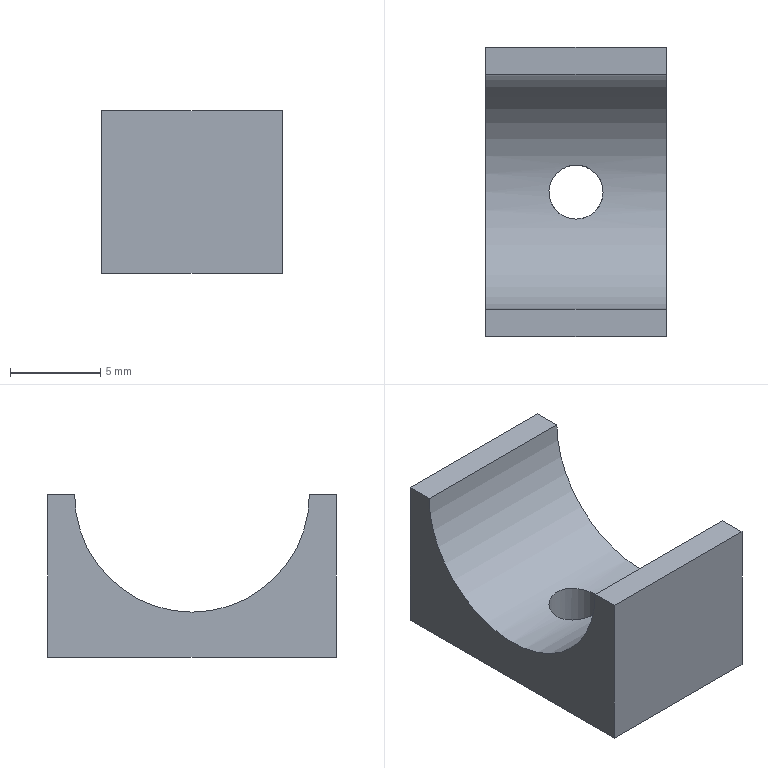Component | NX | 12A__27 | 1 solid | 9 faces | box 10 x 16 x 9 mm | volume 758 mm3 | plane 7 | cylinder 2 | commonest cylinder face diameters 13 x1 3 x1
STEP:
#1=CARTESIAN_POINT('',(0.,0.,0.));
#2=DIRECTION('',(0.,0.,1.));
#3=DIRECTION('',(1.,0.,0.));
#4=AXIS2_PLACEMENT_3D('',#1,#2,#3);
#5=CARTESIAN_POINT('',(34.022,103.108,73.432));
#6=VERTEX_POINT('',#5);
#7=CARTESIAN_POINT('',(44.022,103.108,73.432));
#8=VERTEX_POINT('',#7);
#9=CARTESIAN_POINT('',(34.022,103.108,73.432));
#10=DIRECTION('',(1.,0.,0.));
#11=VECTOR('',#10,1.);
#12=LINE('',#9,#11);
#13=CARTESIAN_POINT('',(34.022,109.608,73.432));
#14=DIRECTION('',(1.,0.,0.));
#15=DIRECTION('',(0.,0.,1.));
#16=AXIS2_PLACEMENT_3D('',#13,#14,#15);
#17=CYLINDRICAL_SURFACE('',#16,6.5);
#18=CARTESIAN_POINT('',(1.571,0.));
#19=DIRECTION('',(0.,1.));
#20=VECTOR('',#19,1.);
#21=LINE('',#18,#20);
#22=(GEOMETRIC_REPRESENTATION_CONTEXT(2)PARAMETRIC_REPRESENTATION_CONTEXT()REPRESENTATION_CONTEXT('',''));
#23=DEFINITIONAL_REPRESENTATION('',(#21),#22);
#24=PCURVE('',#17,#23);
#25=CARTESIAN_POINT('',(34.022,101.608,73.432));
#26=DIRECTION('',(0.,0.,-1.));
#27=DIRECTION('',(1.,0.,0.));
#28=AXIS2_PLACEMENT_3D('',#25,#26,#27);
#29=PLANE('',#28);
#30=CARTESIAN_POINT('',(0.,-1.5));
#31=DIRECTION('',(1.,0.));
#32=VECTOR('',#31,1.);
#33=LINE('',#30,#32);
#34=(GEOMETRIC_REPRESENTATION_CONTEXT(2)PARAMETRIC_REPRESENTATION_CONTEXT()REPRESENTATION_CONTEXT('',''));
#35=DEFINITIONAL_REPRESENTATION('',(#33),#34);
#36=PCURVE('',#29,#35);
#37=SURFACE_CURVE('',#12,(#24,#36),.PCURVE_S1.);
#38=EDGE_CURVE('',#6,#8,#37,.T.);
#39=ORIENTED_EDGE('',*,*,#38,.F.);
#40=CARTESIAN_POINT('',(34.022,116.108,73.432));
#41=VERTEX_POINT('',#40);
#42=CARTESIAN_POINT('',(34.022,109.608,73.432));
#43=DIRECTION('',(1.,0.,0.));
#44=DIRECTION('',(0.,-1.,0.));
#45=AXIS2_PLACEMENT_3D('',#42,#43,#44);
#46=CIRCLE('',#45,6.5);
#47=CARTESIAN_POINT('',(1.571,0.));
#48=DIRECTION('',(1.,0.));
#49=VECTOR('',#48,1.);
#50=LINE('',#47,#49);
#51=(GEOMETRIC_REPRESENTATION_CONTEXT(2)PARAMETRIC_REPRESENTATION_CONTEXT()REPRESENTATION_CONTEXT('',''));
#52=DEFINITIONAL_REPRESENTATION('',(#50),#51);
#53=PCURVE('',#17,#52);
#54=CARTESIAN_POINT('',(34.022,109.608,73.432));
#55=DIRECTION('',(1.,0.,0.));
#56=DIRECTION('',(0.,0.,1.));
#57=AXIS2_PLACEMENT_3D('',#54,#55,#56);
#58=PLANE('',#57);
#59=CARTESIAN_POINT('',(0.,0.));
#60=DIRECTION('',(0.,1.));
#61=AXIS2_PLACEMENT_2D('',#59,#60);
#62=CIRCLE('',#61,6.5);
#63=(GEOMETRIC_REPRESENTATION_CONTEXT(2)PARAMETRIC_REPRESENTATION_CONTEXT()REPRESENTATION_CONTEXT('',''));
#64=DEFINITIONAL_REPRESENTATION('',(#62),#63);
#65=PCURVE('',#58,#64);
#66=SURFACE_CURVE('',#46,(#53,#65),.PCURVE_S1.);
#67=EDGE_CURVE('',#6,#41,#66,.T.);
#68=ORIENTED_EDGE('',*,*,#67,.T.);
#69=CARTESIAN_POINT('',(44.022,116.108,73.432));
#70=VERTEX_POINT('',#69);
#71=CARTESIAN_POINT('',(34.022,116.108,73.432));
#72=DIRECTION('',(1.,0.,0.));
#73=VECTOR('',#72,1.);
#74=LINE('',#71,#73);
#75=CARTESIAN_POINT('',(4.712,0.));
#76=DIRECTION('',(0.,1.));
#77=VECTOR('',#76,1.);
#78=LINE('',#75,#77);
#79=(GEOMETRIC_REPRESENTATION_CONTEXT(2)PARAMETRIC_REPRESENTATION_CONTEXT()REPRESENTATION_CONTEXT('',''));
#80=DEFINITIONAL_REPRESENTATION('',(#78),#79);
#81=PCURVE('',#17,#80);
#82=CARTESIAN_POINT('',(34.022,116.108,73.432));
#83=DIRECTION('',(0.,0.,-1.));
#84=DIRECTION('',(1.,0.,0.));
#85=AXIS2_PLACEMENT_3D('',#82,#83,#84);
#86=PLANE('',#85);
#87=CARTESIAN_POINT('',(0.,0.));
#88=DIRECTION('',(1.,0.));
#89=VECTOR('',#88,1.);
#90=LINE('',#87,#89);
#91=(GEOMETRIC_REPRESENTATION_CONTEXT(2)PARAMETRIC_REPRESENTATION_CONTEXT()REPRESENTATION_CONTEXT('',''));
#92=DEFINITIONAL_REPRESENTATION('',(#90),#91);
#93=PCURVE('',#86,#92);
#94=SURFACE_CURVE('',#74,(#81,#93),.PCURVE_S1.);
#95=EDGE_CURVE('',#41,#70,#94,.T.);
#96=ORIENTED_EDGE('',*,*,#95,.T.);
#97=CARTESIAN_POINT('',(44.022,109.608,73.432));
#98=DIRECTION('',(1.,0.,0.));
#99=DIRECTION('',(0.,1.,0.));
#100=AXIS2_PLACEMENT_3D('',#97,#98,#99);
#101=CIRCLE('',#100,6.5);
#102=CARTESIAN_POINT('',(-1.571,10.));
#103=DIRECTION('',(1.,0.));
#104=VECTOR('',#103,1.);
#105=LINE('',#102,#104);
#106=(GEOMETRIC_REPRESENTATION_CONTEXT(2)PARAMETRIC_REPRESENTATION_CONTEXT()REPRESENTATION_CONTEXT('',''));
#107=DEFINITIONAL_REPRESENTATION('',(#105),#106);
#108=PCURVE('',#17,#107);
#109=CARTESIAN_POINT('',(44.022,109.608,73.432));
#110=DIRECTION('',(1.,0.,0.));
#111=DIRECTION('',(0.,0.,1.));
#112=AXIS2_PLACEMENT_3D('',#109,#110,#111);
#113=PLANE('',#112);
#114=CARTESIAN_POINT('',(0.,0.));
#115=DIRECTION('',(0.,-1.));
#116=AXIS2_PLACEMENT_2D('',#114,#115);
#117=CIRCLE('',#116,6.5);
#118=(GEOMETRIC_REPRESENTATION_CONTEXT(2)PARAMETRIC_REPRESENTATION_CONTEXT()REPRESENTATION_CONTEXT('',''));
#119=DEFINITIONAL_REPRESENTATION('',(#117),#118);
#120=PCURVE('',#113,#119);
#121=SURFACE_CURVE('',#101,(#108,#120),.PCURVE_S1.);
#122=EDGE_CURVE('',#8,#70,#121,.T.);
#123=ORIENTED_EDGE('',*,*,#122,.F.);
#124=EDGE_LOOP('',(#39,#68,#96,#123));
#125=FACE_BOUND('',#124,.F.);
#126=CARTESIAN_POINT('',(40.522,109.608,66.932));
#127=VERTEX_POINT('',#126);
#128=CARTESIAN_POINT('',(40.522,109.608,66.932));
#129=CARTESIAN_POINT('',(40.522,109.774,66.932));
#130=CARTESIAN_POINT('',(40.494,109.941,66.938));
#131=CARTESIAN_POINT('',(40.44,110.097,66.95));
#132=CARTESIAN_POINT('',(40.386,110.253,66.962));
#133=CARTESIAN_POINT('',(40.306,110.402,66.979));
#134=CARTESIAN_POINT('',(40.204,110.531,66.998));
#135=CARTESIAN_POINT('',(40.102,110.663,67.016));
#136=CARTESIAN_POINT('',(39.975,110.778,67.037));
#137=CARTESIAN_POINT('',(39.835,110.869,67.055));
#138=CARTESIAN_POINT('',(39.693,110.96,67.073));
#139=CARTESIAN_POINT('',(39.532,111.029,67.089));
#140=CARTESIAN_POINT('',(39.367,111.068,67.098));
#141=CARTESIAN_POINT('',(39.205,111.106,67.107));
#142=CARTESIAN_POINT('',(39.033,111.117,67.109));
#143=CARTESIAN_POINT('',(38.867,111.1,67.105));
#144=CARTESIAN_POINT('',(38.704,111.083,67.101));
#145=CARTESIAN_POINT('',(38.542,111.039,67.091));
#146=CARTESIAN_POINT('',(38.394,110.97,67.076));
#147=CARTESIAN_POINT('',(38.245,110.902,67.061));
#148=CARTESIAN_POINT('',(38.106,110.807,67.042));
#149=CARTESIAN_POINT('',(37.987,110.694,67.023));
#150=CARTESIAN_POINT('',(37.865,110.578,67.003));
#151=CARTESIAN_POINT('',(37.762,110.439,66.983));
#152=CARTESIAN_POINT('',(37.686,110.289,66.967));
#153=CARTESIAN_POINT('',(37.609,110.139,66.952));
#154=CARTESIAN_POINT('',(37.557,109.972,66.94));
#155=CARTESIAN_POINT('',(37.535,109.804,66.935));
#156=CARTESIAN_POINT('',(37.513,109.64,66.93));
#157=CARTESIAN_POINT('',(37.519,109.47,66.931));
#158=CARTESIAN_POINT('',(37.553,109.307,66.939));
#159=CARTESIAN_POINT('',(37.585,109.147,66.946));
#160=CARTESIAN_POINT('',(37.646,108.99,66.96));
#161=CARTESIAN_POINT('',(37.728,108.85,66.976));
#162=CARTESIAN_POINT('',(37.812,108.707,66.993));
#163=CARTESIAN_POINT('',(37.92,108.577,67.013));
#164=CARTESIAN_POINT('',(38.046,108.469,67.032));
#165=CARTESIAN_POINT('',(38.174,108.359,67.052));
#166=CARTESIAN_POINT('',(38.323,108.27,67.071));
#167=CARTESIAN_POINT('',(38.481,108.209,67.084));
#168=CARTESIAN_POINT('',(38.638,108.148,67.097));
#169=CARTESIAN_POINT('',(38.808,108.114,67.106));
#170=CARTESIAN_POINT('',(38.976,108.109,67.107));
#171=CARTESIAN_POINT('',(39.141,108.104,67.108));
#172=CARTESIAN_POINT('',(39.309,108.127,67.103));
#173=CARTESIAN_POINT('',(39.466,108.175,67.092));
#174=CARTESIAN_POINT('',(39.622,108.223,67.081));
#175=CARTESIAN_POINT('',(39.772,108.299,67.064));
#176=CARTESIAN_POINT('',(39.904,108.394,67.046));
#177=CARTESIAN_POINT('',(40.038,108.492,67.027));
#178=CARTESIAN_POINT('',(40.158,108.614,67.007));
#179=CARTESIAN_POINT('',(40.253,108.751,66.988));
#180=CARTESIAN_POINT('',(40.35,108.89,66.97));
#181=CARTESIAN_POINT('',(40.424,109.048,66.954));
#182=CARTESIAN_POINT('',(40.469,109.211,66.944));
#183=CARTESIAN_POINT('',(40.504,109.34,66.936));
#184=CARTESIAN_POINT('',(40.522,109.475,66.932));
#185=CARTESIAN_POINT('',(40.522,109.608,66.932));
#186=B_SPLINE_CURVE_WITH_KNOTS('',3,(#128,#129,#130,#131,#132,#133,#134,#135,#136,#137,#138,#139,#140,#141,#142,#143,#144,#145,#146,#147,#148,#149,#150,#151,#152,#153,#154,#155,#156,#157,#158,#159,#160,#161,#162,#163,#164,#165,#166,#167,#168,#169,#170,#171,#172,#173,#174,#175,#176,#177,#178,#179,#180,#181,#182,#183,#184,#185),.UNSPECIFIED.,.T.,.F.,(1,3,3,3,3,3,3,3,3,3,3,3,3,3,3,3,3,3,3,3,3,1),(-0.04234,0.,0.05275,0.1054,0.159,0.2132,0.2665,0.3187,0.3713,0.4252,0.4793,0.5321,0.5843,0.6373,0.6915,0.7453,0.7978,0.85,0.9034,0.9577,1.,1.053),.UNSPECIFIED.);
#187=CARTESIAN_POINT('',(3.142,6.5));
#188=CARTESIAN_POINT('',(3.147,6.5));
#189=CARTESIAN_POINT('',(3.158,6.497));
#190=CARTESIAN_POINT('',(3.175,6.486));
#191=CARTESIAN_POINT('',(3.191,6.467));
#192=CARTESIAN_POINT('',(3.207,6.44));
#193=CARTESIAN_POINT('',(3.223,6.406));
#194=CARTESIAN_POINT('',(3.238,6.365));
#195=CARTESIAN_POINT('',(3.253,6.317));
#196=CARTESIAN_POINT('',(3.267,6.262));
#197=CARTESIAN_POINT('',(3.281,6.201));
#198=CARTESIAN_POINT('',(3.293,6.135));
#199=CARTESIAN_POINT('',(3.306,6.062));
#200=CARTESIAN_POINT('',(3.317,5.983));
#201=CARTESIAN_POINT('',(3.328,5.9));
#202=CARTESIAN_POINT('',(3.337,5.813));
#203=CARTESIAN_POINT('',(3.346,5.721));
#204=CARTESIAN_POINT('',(3.353,5.625));
#205=CARTESIAN_POINT('',(3.36,5.526));
#206=CARTESIAN_POINT('',(3.365,5.424));
#207=CARTESIAN_POINT('',(3.369,5.321));
#208=CARTESIAN_POINT('',(3.372,5.215));
#209=CARTESIAN_POINT('',(3.374,5.108));
#210=CARTESIAN_POINT('',(3.375,5.));
#211=CARTESIAN_POINT('',(3.374,4.893));
#212=CARTESIAN_POINT('',(3.372,4.787));
#213=CARTESIAN_POINT('',(3.369,4.681));
#214=CARTESIAN_POINT('',(3.365,4.576));
#215=CARTESIAN_POINT('',(3.36,4.474));
#216=CARTESIAN_POINT('',(3.353,4.376));
#217=CARTESIAN_POINT('',(3.346,4.28));
#218=CARTESIAN_POINT('',(3.337,4.188));
#219=CARTESIAN_POINT('',(3.328,4.1));
#220=CARTESIAN_POINT('',(3.317,4.017));
#221=CARTESIAN_POINT('',(3.306,3.939));
#222=CARTESIAN_POINT('',(3.294,3.866));
#223=CARTESIAN_POINT('',(3.281,3.799));
#224=CARTESIAN_POINT('',(3.267,3.738));
#225=CARTESIAN_POINT('',(3.253,3.683));
#226=CARTESIAN_POINT('',(3.238,3.635));
#227=CARTESIAN_POINT('',(3.223,3.594));
#228=CARTESIAN_POINT('',(3.207,3.56));
#229=CARTESIAN_POINT('',(3.191,3.533));
#230=CARTESIAN_POINT('',(3.175,3.514));
#231=CARTESIAN_POINT('',(3.158,3.503));
#232=CARTESIAN_POINT('',(3.142,3.499));
#233=CARTESIAN_POINT('',(3.125,3.503));
#234=CARTESIAN_POINT('',(3.109,3.514));
#235=CARTESIAN_POINT('',(3.092,3.533));
#236=CARTESIAN_POINT('',(3.076,3.56));
#237=CARTESIAN_POINT('',(3.061,3.594));
#238=CARTESIAN_POINT('',(3.045,3.635));
#239=CARTESIAN_POINT('',(3.031,3.683));
#240=CARTESIAN_POINT('',(3.016,3.737));
#241=CARTESIAN_POINT('',(3.003,3.798));
#242=CARTESIAN_POINT('',(2.99,3.865));
#243=CARTESIAN_POINT('',(2.978,3.938));
#244=CARTESIAN_POINT('',(2.966,4.016));
#245=CARTESIAN_POINT('',(2.956,4.099));
#246=CARTESIAN_POINT('',(2.946,4.187));
#247=CARTESIAN_POINT('',(2.938,4.279));
#248=CARTESIAN_POINT('',(2.93,4.375));
#249=CARTESIAN_POINT('',(2.924,4.473));
#250=CARTESIAN_POINT('',(2.918,4.575));
#251=CARTESIAN_POINT('',(2.914,4.679));
#252=CARTESIAN_POINT('',(2.911,4.785));
#253=CARTESIAN_POINT('',(2.909,4.892));
#254=CARTESIAN_POINT('',(2.909,4.999));
#255=CARTESIAN_POINT('',(2.909,5.106));
#256=CARTESIAN_POINT('',(2.911,5.213));
#257=CARTESIAN_POINT('',(2.914,5.319));
#258=CARTESIAN_POINT('',(2.918,5.423));
#259=CARTESIAN_POINT('',(2.923,5.524));
#260=CARTESIAN_POINT('',(2.93,5.624));
#261=CARTESIAN_POINT('',(2.937,5.72));
#262=CARTESIAN_POINT('',(2.946,5.812));
#263=CARTESIAN_POINT('',(2.956,5.899));
#264=CARTESIAN_POINT('',(2.966,5.982));
#265=CARTESIAN_POINT('',(2.977,6.061));
#266=CARTESIAN_POINT('',(2.99,6.134));
#267=CARTESIAN_POINT('',(3.003,6.201));
#268=CARTESIAN_POINT('',(3.016,6.262));
#269=CARTESIAN_POINT('',(3.03,6.316));
#270=CARTESIAN_POINT('',(3.045,6.364));
#271=CARTESIAN_POINT('',(3.06,6.406));
#272=CARTESIAN_POINT('',(3.076,6.44));
#273=CARTESIAN_POINT('',(3.092,6.466));
#274=CARTESIAN_POINT('',(3.109,6.486));
#275=CARTESIAN_POINT('',(3.125,6.497));
#276=CARTESIAN_POINT('',(3.136,6.5));
#277=CARTESIAN_POINT('',(3.142,6.5));
#278=B_SPLINE_CURVE_WITH_KNOTS('',3,(#187,#188,#189,#190,#191,#192,#193,#194,#195,#196,#197,#198,#199,#200,#201,#202,#203,#204,#205,#206,#207,#208,#209,#210,#211,#212,#213,#214,#215,#216,#217,#218,#219,#220,#221,#222,#223,#224,#225,#226,#227,#228,#229,#230,#231,#232,#233,#234,#235,#236,#237,#238,#239,#240,#241,#242,#243,#244,#245,#246,#247,#248,#249,#250,#251,#252,#253,#254,#255,#256,#257,#258,#259,#260,#261,#262,#263,#264,#265,#266,#267,#268,#269,#270,#271,#272,#273,#274,#275,#276,#277),.UNSPECIFIED.,.T.,.F.,(4,1,1,1,1,1,1,1,1,1,1,1,1,1,1,1,1,1,1,1,1,1,1,1,1,1,1,1,1,1,1,1,1,1,1,1,1,1,1,1,1,1,1,1,1,1,1,1,1,1,1,1,1,1,1,1,1,1,1,1,1,1,1,1,1,1,1,1,1,1,1,1,1,1,1,1,1,1,1,1,1,1,1,1,1,1,1,1,4),(0.,0.01136,0.02273,0.03409,0.04545,0.05682,0.06818,0.07955,0.09091,0.1023,0.1136,0.125,0.1364,0.1477,0.1591,0.1705,0.1818,0.1932,0.2045,0.2159,0.2273,0.2386,0.25,0.2614,0.2727,0.2841,0.2955,0.3068,0.3182,0.3295,0.3409,0.3523,0.3636,0.375,0.3864,0.3977,0.4091,0.4205,0.4318,0.4432,0.4545,0.4659,0.4773,0.4886,0.5,0.5114,0.5227,0.5341,0.5455,0.5568,0.5682,0.5795,0.5909,0.6023,0.6136,0.625,0.6364,0.6477,0.6591,0.6705,0.6818,0.6932,0.7045,0.7159,0.7273,0.7386,0.75,0.7614,0.7727,0.7841,0.7955,0.8068,0.8182,0.8295,0.8409,0.8523,0.8636,0.875,0.8864,0.8977,0.9091,0.9205,0.9318,0.9432,0.9545,0.9659,0.9773,0.9886,1.),.QUASI_UNIFORM_KNOTS.);
#279=(GEOMETRIC_REPRESENTATION_CONTEXT(2)PARAMETRIC_REPRESENTATION_CONTEXT()REPRESENTATION_CONTEXT('',''));
#280=DEFINITIONAL_REPRESENTATION('',(#278),#279);
#281=PCURVE('',#17,#280);
#282=CARTESIAN_POINT('',(39.022,109.608,74.432));
#283=DIRECTION('',(0.,0.,-1.));
#284=DIRECTION('',(1.,0.,0.));
#285=AXIS2_PLACEMENT_3D('',#282,#283,#284);
#286=CYLINDRICAL_SURFACE('',#285,1.5);
#287=CARTESIAN_POINT('',(6.283,7.5));
#288=CARTESIAN_POINT('',(6.259,7.5));
#289=CARTESIAN_POINT('',(6.212,7.499));
#290=CARTESIAN_POINT('',(6.14,7.497));
#291=CARTESIAN_POINT('',(6.068,7.492));
#292=CARTESIAN_POINT('',(5.997,7.486));
#293=CARTESIAN_POINT('',(5.926,7.479));
#294=CARTESIAN_POINT('',(5.854,7.47));
#295=CARTESIAN_POINT('',(5.783,7.46));
#296=CARTESIAN_POINT('',(5.711,7.449));
#297=CARTESIAN_POINT('',(5.64,7.438));
#298=CARTESIAN_POINT('',(5.569,7.425));
#299=CARTESIAN_POINT('',(5.498,7.413));
#300=CARTESIAN_POINT('',(5.427,7.4));
#301=CARTESIAN_POINT('',(5.355,7.388));
#302=CARTESIAN_POINT('',(5.284,7.376));
#303=CARTESIAN_POINT('',(5.213,7.365));
#304=CARTESIAN_POINT('',(5.142,7.355));
#305=CARTESIAN_POINT('',(5.07,7.346));
#306=CARTESIAN_POINT('',(4.999,7.338));
#307=CARTESIAN_POINT('',(4.928,7.332));
#308=CARTESIAN_POINT('',(4.856,7.328));
#309=CARTESIAN_POINT('',(4.784,7.325));
#310=CARTESIAN_POINT('',(4.713,7.324));
#311=CARTESIAN_POINT('',(4.641,7.325));
#312=CARTESIAN_POINT('',(4.57,7.328));
#313=CARTESIAN_POINT('',(4.498,7.332));
#314=CARTESIAN_POINT('',(4.426,7.339));
#315=CARTESIAN_POINT('',(4.355,7.346));
#316=CARTESIAN_POINT('',(4.283,7.355));
#317=CARTESIAN_POINT('',(4.212,7.365));
#318=CARTESIAN_POINT('',(4.141,7.376));
#319=CARTESIAN_POINT('',(4.07,7.388));
#320=CARTESIAN_POINT('',(3.998,7.4));
#321=CARTESIAN_POINT('',(3.927,7.413));
#322=CARTESIAN_POINT('',(3.856,7.425));
#323=CARTESIAN_POINT('',(3.785,7.437));
#324=CARTESIAN_POINT('',(3.714,7.449));
#325=CARTESIAN_POINT('',(3.642,7.46));
#326=CARTESIAN_POINT('',(3.571,7.47));
#327=CARTESIAN_POINT('',(3.5,7.479));
#328=CARTESIAN_POINT('',(3.428,7.486));
#329=CARTESIAN_POINT('',(3.357,7.492));
#330=CARTESIAN_POINT('',(3.285,7.497));
#331=CARTESIAN_POINT('',(3.214,7.499));
#332=CARTESIAN_POINT('',(3.142,7.5));
#333=CARTESIAN_POINT('',(3.07,7.499));
#334=CARTESIAN_POINT('',(2.999,7.497));
#335=CARTESIAN_POINT('',(2.927,7.492));
#336=CARTESIAN_POINT('',(2.856,7.486));
#337=CARTESIAN_POINT('',(2.784,7.479));
#338=CARTESIAN_POINT('',(2.713,7.47));
#339=CARTESIAN_POINT('',(2.641,7.46));
#340=CARTESIAN_POINT('',(2.57,7.449));
#341=CARTESIAN_POINT('',(2.499,7.438));
#342=CARTESIAN_POINT('',(2.428,7.425));
#343=CARTESIAN_POINT('',(2.357,7.413));
#344=CARTESIAN_POINT('',(2.285,7.4));
#345=CARTESIAN_POINT('',(2.215,7.388));
#346=CARTESIAN_POINT('',(2.143,7.376));
#347=CARTESIAN_POINT('',(2.072,7.365));
#348=CARTESIAN_POINT('',(2.,7.355));
#349=CARTESIAN_POINT('',(1.929,7.346));
#350=CARTESIAN_POINT('',(1.858,7.339));
#351=CARTESIAN_POINT('',(1.786,7.332));
#352=CARTESIAN_POINT('',(1.715,7.328));
#353=CARTESIAN_POINT('',(1.643,7.325));
#354=CARTESIAN_POINT('',(1.572,7.324));
#355=CARTESIAN_POINT('',(1.5,7.325));
#356=CARTESIAN_POINT('',(1.428,7.328));
#357=CARTESIAN_POINT('',(1.357,7.332));
#358=CARTESIAN_POINT('',(1.285,7.338));
#359=CARTESIAN_POINT('',(1.214,7.346));
#360=CARTESIAN_POINT('',(1.142,7.355));
#361=CARTESIAN_POINT('',(1.071,7.365));
#362=CARTESIAN_POINT('',(0.9995,7.376));
#363=CARTESIAN_POINT('',(0.9286,7.388));
#364=CARTESIAN_POINT('',(0.8575,7.4));
#365=CARTESIAN_POINT('',(0.7862,7.413));
#366=CARTESIAN_POINT('',(0.7149,7.425));
#367=CARTESIAN_POINT('',(0.6436,7.437));
#368=CARTESIAN_POINT('',(0.5728,7.449));
#369=CARTESIAN_POINT('',(0.5015,7.46));
#370=CARTESIAN_POINT('',(0.43,7.47));
#371=CARTESIAN_POINT('',(0.3585,7.479));
#372=CARTESIAN_POINT('',(0.2872,7.486));
#373=CARTESIAN_POINT('',(0.2157,7.492));
#374=CARTESIAN_POINT('',(0.1438,7.497));
#375=CARTESIAN_POINT('',(0.07178,7.499));
#376=CARTESIAN_POINT('',(0.02388,7.5));
#377=CARTESIAN_POINT('',(0.,7.5));
#378=B_SPLINE_CURVE_WITH_KNOTS('',3,(#287,#288,#289,#290,#291,#292,#293,#294,#295,#296,#297,#298,#299,#300,#301,#302,#303,#304,#305,#306,#307,#308,#309,#310,#311,#312,#313,#314,#315,#316,#317,#318,#319,#320,#321,#322,#323,#324,#325,#326,#327,#328,#329,#330,#331,#332,#333,#334,#335,#336,#337,#338,#339,#340,#341,#342,#343,#344,#345,#346,#347,#348,#349,#350,#351,#352,#353,#354,#355,#356,#357,#358,#359,#360,#361,#362,#363,#364,#365,#366,#367,#368,#369,#370,#371,#372,#373,#374,#375,#376,#377),.UNSPECIFIED.,.F.,.F.,(4,1,1,1,1,1,1,1,1,1,1,1,1,1,1,1,1,1,1,1,1,1,1,1,1,1,1,1,1,1,1,1,1,1,1,1,1,1,1,1,1,1,1,1,1,1,1,1,1,1,1,1,1,1,1,1,1,1,1,1,1,1,1,1,1,1,1,1,1,1,1,1,1,1,1,1,1,1,1,1,1,1,1,1,1,1,1,1,4),(0.,0.01136,0.02273,0.03409,0.04545,0.05682,0.06818,0.07955,0.09091,0.1023,0.1136,0.125,0.1364,0.1477,0.1591,0.1705,0.1818,0.1932,0.2045,0.2159,0.2273,0.2386,0.25,0.2614,0.2727,0.2841,0.2955,0.3068,0.3182,0.3295,0.3409,0.3523,0.3636,0.375,0.3864,0.3977,0.4091,0.4205,0.4318,0.4432,0.4545,0.4659,0.4773,0.4886,0.5,0.5114,0.5227,0.5341,0.5455,0.5568,0.5682,0.5795,0.5909,0.6023,0.6136,0.625,0.6364,0.6477,0.6591,0.6705,0.6818,0.6932,0.7045,0.7159,0.7273,0.7386,0.75,0.7614,0.7727,0.7841,0.7955,0.8068,0.8182,0.8295,0.8409,0.8523,0.8636,0.875,0.8864,0.8977,0.9091,0.9205,0.9318,0.9432,0.9545,0.9659,0.9773,0.9886,1.),.QUASI_UNIFORM_KNOTS.);
#379=(GEOMETRIC_REPRESENTATION_CONTEXT(2)PARAMETRIC_REPRESENTATION_CONTEXT()REPRESENTATION_CONTEXT('',''));
#380=DEFINITIONAL_REPRESENTATION('',(#378),#379);
#381=PCURVE('',#286,#380);
#382=SURFACE_CURVE('',#186,(#281,#381),.PCURVE_S1.);
#383=EDGE_CURVE('',#127,#127,#382,.T.);
#384=ORIENTED_EDGE('',*,*,#383,.T.);
#385=EDGE_LOOP('',(#384));
#386=FACE_BOUND('',#385,.F.);
#387=ADVANCED_FACE('',(#125,#386),#17,.F.);
#388=CARTESIAN_POINT('',(44.022,101.608,64.432));
#389=VERTEX_POINT('',#388);
#390=CARTESIAN_POINT('',(44.022,101.608,73.432));
#391=VERTEX_POINT('',#390);
#392=CARTESIAN_POINT('',(44.022,101.608,64.432));
#393=DIRECTION('',(0.,0.,1.));
#394=VECTOR('',#393,1.);
#395=LINE('',#392,#394);
#396=CARTESIAN_POINT('',(34.022,101.608,64.432));
#397=DIRECTION('',(0.,1.,0.));
#398=DIRECTION('',(0.,0.,-1.));
#399=AXIS2_PLACEMENT_3D('',#396,#397,#398);
#400=PLANE('',#399);
#401=CARTESIAN_POINT('',(0.,-10.));
#402=DIRECTION('',(-1.,0.));
#403=VECTOR('',#402,1.);
#404=LINE('',#401,#403);
#405=(GEOMETRIC_REPRESENTATION_CONTEXT(2)PARAMETRIC_REPRESENTATION_CONTEXT()REPRESENTATION_CONTEXT('',''));
#406=DEFINITIONAL_REPRESENTATION('',(#404),#405);
#407=PCURVE('',#400,#406);
#408=CARTESIAN_POINT('',(-9.,8.));
#409=DIRECTION('',(1.,0.));
#410=VECTOR('',#409,1.);
#411=LINE('',#408,#410);
#412=(GEOMETRIC_REPRESENTATION_CONTEXT(2)PARAMETRIC_REPRESENTATION_CONTEXT()REPRESENTATION_CONTEXT('',''));
#413=DEFINITIONAL_REPRESENTATION('',(#411),#412);
#414=PCURVE('',#113,#413);
#415=SURFACE_CURVE('',#395,(#407,#414),.PCURVE_S1.);
#416=EDGE_CURVE('',#389,#391,#415,.T.);
#417=ORIENTED_EDGE('',*,*,#416,.T.);
#418=CARTESIAN_POINT('',(34.022,101.608,73.432));
#419=VERTEX_POINT('',#418);
#420=CARTESIAN_POINT('',(34.022,101.608,73.432));
#421=DIRECTION('',(1.,0.,0.));
#422=VECTOR('',#421,1.);
#423=LINE('',#420,#422);
#424=CARTESIAN_POINT('',(-9.,0.));
#425=DIRECTION('',(0.,-1.));
#426=VECTOR('',#425,1.);
#427=LINE('',#424,#426);
#428=(GEOMETRIC_REPRESENTATION_CONTEXT(2)PARAMETRIC_REPRESENTATION_CONTEXT()REPRESENTATION_CONTEXT('',''));
#429=DEFINITIONAL_REPRESENTATION('',(#427),#428);
#430=PCURVE('',#400,#429);
#431=CARTESIAN_POINT('',(0.,0.));
#432=DIRECTION('',(1.,0.));
#433=VECTOR('',#432,1.);
#434=LINE('',#431,#433);
#435=(GEOMETRIC_REPRESENTATION_CONTEXT(2)PARAMETRIC_REPRESENTATION_CONTEXT()REPRESENTATION_CONTEXT('',''));
#436=DEFINITIONAL_REPRESENTATION('',(#434),#435);
#437=PCURVE('',#29,#436);
#438=SURFACE_CURVE('',#423,(#430,#437),.PCURVE_S1.);
#439=EDGE_CURVE('',#419,#391,#438,.T.);
#440=ORIENTED_EDGE('',*,*,#439,.F.);
#441=CARTESIAN_POINT('',(34.022,101.608,64.432));
#442=VERTEX_POINT('',#441);
#443=CARTESIAN_POINT('',(34.022,101.608,64.432));
#444=DIRECTION('',(0.,0.,1.));
#445=VECTOR('',#444,1.);
#446=LINE('',#443,#445);
#447=CARTESIAN_POINT('',(0.,0.));
#448=DIRECTION('',(-1.,0.));
#449=VECTOR('',#448,1.);
#450=LINE('',#447,#449);
#451=(GEOMETRIC_REPRESENTATION_CONTEXT(2)PARAMETRIC_REPRESENTATION_CONTEXT()REPRESENTATION_CONTEXT('',''));
#452=DEFINITIONAL_REPRESENTATION('',(#450),#451);
#453=PCURVE('',#400,#452);
#454=CARTESIAN_POINT('',(-9.,8.));
#455=DIRECTION('',(1.,0.));
#456=VECTOR('',#455,1.);
#457=LINE('',#454,#456);
#458=(GEOMETRIC_REPRESENTATION_CONTEXT(2)PARAMETRIC_REPRESENTATION_CONTEXT()REPRESENTATION_CONTEXT('',''));
#459=DEFINITIONAL_REPRESENTATION('',(#457),#458);
#460=PCURVE('',#58,#459);
#461=SURFACE_CURVE('',#446,(#453,#460),.PCURVE_S1.);
#462=EDGE_CURVE('',#442,#419,#461,.T.);
#463=ORIENTED_EDGE('',*,*,#462,.F.);
#464=CARTESIAN_POINT('',(34.022,101.608,64.432));
#465=DIRECTION('',(1.,0.,0.));
#466=VECTOR('',#465,1.);
#467=LINE('',#464,#466);
#468=CARTESIAN_POINT('',(0.,0.));
#469=DIRECTION('',(0.,-1.));
#470=VECTOR('',#469,1.);
#471=LINE('',#468,#470);
#472=(GEOMETRIC_REPRESENTATION_CONTEXT(2)PARAMETRIC_REPRESENTATION_CONTEXT()REPRESENTATION_CONTEXT('',''));
#473=DEFINITIONAL_REPRESENTATION('',(#471),#472);
#474=PCURVE('',#400,#473);
#475=CARTESIAN_POINT('',(34.022,117.608,64.432));
#476=DIRECTION('',(0.,0.,1.));
#477=DIRECTION('',(-1.,0.,0.));
#478=AXIS2_PLACEMENT_3D('',#475,#476,#477);
#479=PLANE('',#478);
#480=CARTESIAN_POINT('',(0.,16.));
#481=DIRECTION('',(-1.,0.));
#482=VECTOR('',#481,1.);
#483=LINE('',#480,#482);
#484=(GEOMETRIC_REPRESENTATION_CONTEXT(2)PARAMETRIC_REPRESENTATION_CONTEXT()REPRESENTATION_CONTEXT('',''));
#485=DEFINITIONAL_REPRESENTATION('',(#483),#484);
#486=PCURVE('',#479,#485);
#487=SURFACE_CURVE('',#467,(#474,#486),.PCURVE_S1.);
#488=EDGE_CURVE('',#442,#389,#487,.T.);
#489=ORIENTED_EDGE('',*,*,#488,.T.);
#490=EDGE_LOOP('',(#417,#440,#463,#489));
#491=FACE_BOUND('',#490,.T.);
#492=ADVANCED_FACE('',(#491),#400,.F.);
#493=CARTESIAN_POINT('',(44.022,101.608,73.432));
#494=DIRECTION('',(0.,1.,0.));
#495=VECTOR('',#494,1.);
#496=LINE('',#493,#495);
#497=CARTESIAN_POINT('',(10.,0.));
#498=DIRECTION('',(0.,-1.));
#499=VECTOR('',#498,1.);
#500=LINE('',#497,#499);
#501=(GEOMETRIC_REPRESENTATION_CONTEXT(2)PARAMETRIC_REPRESENTATION_CONTEXT()REPRESENTATION_CONTEXT('',''));
#502=DEFINITIONAL_REPRESENTATION('',(#500),#501);
#503=PCURVE('',#29,#502);
#504=CARTESIAN_POINT('',(0.,8.));
#505=DIRECTION('',(0.,-1.));
#506=VECTOR('',#505,1.);
#507=LINE('',#504,#506);
#508=(GEOMETRIC_REPRESENTATION_CONTEXT(2)PARAMETRIC_REPRESENTATION_CONTEXT()REPRESENTATION_CONTEXT('',''));
#509=DEFINITIONAL_REPRESENTATION('',(#507),#508);
#510=PCURVE('',#113,#509);
#511=SURFACE_CURVE('',#496,(#503,#510),.PCURVE_S1.);
#512=EDGE_CURVE('',#391,#8,#511,.T.);
#513=ORIENTED_EDGE('',*,*,#512,.T.);
#514=ORIENTED_EDGE('',*,*,#38,.F.);
#515=CARTESIAN_POINT('',(34.022,101.608,73.432));
#516=DIRECTION('',(0.,1.,0.));
#517=VECTOR('',#516,1.);
#518=LINE('',#515,#517);
#519=CARTESIAN_POINT('',(0.,0.));
#520=DIRECTION('',(0.,-1.));
#521=VECTOR('',#520,1.);
#522=LINE('',#519,#521);
#523=(GEOMETRIC_REPRESENTATION_CONTEXT(2)PARAMETRIC_REPRESENTATION_CONTEXT()REPRESENTATION_CONTEXT('',''));
#524=DEFINITIONAL_REPRESENTATION('',(#522),#523);
#525=PCURVE('',#29,#524);
#526=CARTESIAN_POINT('',(0.,8.));
#527=DIRECTION('',(0.,-1.));
#528=VECTOR('',#527,1.);
#529=LINE('',#526,#528);
#530=(GEOMETRIC_REPRESENTATION_CONTEXT(2)PARAMETRIC_REPRESENTATION_CONTEXT()REPRESENTATION_CONTEXT('',''));
#531=DEFINITIONAL_REPRESENTATION('',(#529),#530);
#532=PCURVE('',#58,#531);
#533=SURFACE_CURVE('',#518,(#525,#532),.PCURVE_S1.);
#534=EDGE_CURVE('',#419,#6,#533,.T.);
#535=ORIENTED_EDGE('',*,*,#534,.F.);
#536=ORIENTED_EDGE('',*,*,#439,.T.);
#537=EDGE_LOOP('',(#513,#514,#535,#536));
#538=FACE_BOUND('',#537,.T.);
#539=ADVANCED_FACE('',(#538),#29,.F.);
#540=CARTESIAN_POINT('',(44.022,117.608,73.432));
#541=VERTEX_POINT('',#540);
#542=CARTESIAN_POINT('',(44.022,116.108,73.432));
#543=DIRECTION('',(0.,1.,0.));
#544=VECTOR('',#543,1.);
#545=LINE('',#542,#544);
#546=CARTESIAN_POINT('',(10.,0.));
#547=DIRECTION('',(0.,-1.));
#548=VECTOR('',#547,1.);
#549=LINE('',#546,#548);
#550=(GEOMETRIC_REPRESENTATION_CONTEXT(2)PARAMETRIC_REPRESENTATION_CONTEXT()REPRESENTATION_CONTEXT('',''));
#551=DEFINITIONAL_REPRESENTATION('',(#549),#550);
#552=PCURVE('',#86,#551);
#553=CARTESIAN_POINT('',(0.,-6.5));
#554=DIRECTION('',(0.,-1.));
#555=VECTOR('',#554,1.);
#556=LINE('',#553,#555);
#557=(GEOMETRIC_REPRESENTATION_CONTEXT(2)PARAMETRIC_REPRESENTATION_CONTEXT()REPRESENTATION_CONTEXT('',''));
#558=DEFINITIONAL_REPRESENTATION('',(#556),#557);
#559=PCURVE('',#113,#558);
#560=SURFACE_CURVE('',#545,(#552,#559),.PCURVE_S1.);
#561=EDGE_CURVE('',#70,#541,#560,.T.);
#562=ORIENTED_EDGE('',*,*,#561,.T.);
#563=CARTESIAN_POINT('',(34.022,117.608,73.432));
#564=VERTEX_POINT('',#563);
#565=CARTESIAN_POINT('',(34.022,117.608,73.432));
#566=DIRECTION('',(1.,0.,0.));
#567=VECTOR('',#566,1.);
#568=LINE('',#565,#567);
#569=CARTESIAN_POINT('',(0.,-1.5));
#570=DIRECTION('',(1.,0.));
#571=VECTOR('',#570,1.);
#572=LINE('',#569,#571);
#573=(GEOMETRIC_REPRESENTATION_CONTEXT(2)PARAMETRIC_REPRESENTATION_CONTEXT()REPRESENTATION_CONTEXT('',''));
#574=DEFINITIONAL_REPRESENTATION('',(#572),#573);
#575=PCURVE('',#86,#574);
#576=CARTESIAN_POINT('',(34.022,117.608,73.432));
#577=DIRECTION('',(0.,-1.,0.));
#578=DIRECTION('',(0.,0.,1.));
#579=AXIS2_PLACEMENT_3D('',#576,#577,#578);
#580=PLANE('',#579);
#581=CARTESIAN_POINT('',(0.,0.));
#582=DIRECTION('',(0.,-1.));
#583=VECTOR('',#582,1.);
#584=LINE('',#581,#583);
#585=(GEOMETRIC_REPRESENTATION_CONTEXT(2)PARAMETRIC_REPRESENTATION_CONTEXT()REPRESENTATION_CONTEXT('',''));
#586=DEFINITIONAL_REPRESENTATION('',(#584),#585);
#587=PCURVE('',#580,#586);
#588=SURFACE_CURVE('',#568,(#575,#587),.PCURVE_S1.);
#589=EDGE_CURVE('',#564,#541,#588,.T.);
#590=ORIENTED_EDGE('',*,*,#589,.F.);
#591=CARTESIAN_POINT('',(34.022,116.108,73.432));
#592=DIRECTION('',(0.,1.,0.));
#593=VECTOR('',#592,1.);
#594=LINE('',#591,#593);
#595=CARTESIAN_POINT('',(0.,0.));
#596=DIRECTION('',(0.,-1.));
#597=VECTOR('',#596,1.);
#598=LINE('',#595,#597);
#599=(GEOMETRIC_REPRESENTATION_CONTEXT(2)PARAMETRIC_REPRESENTATION_CONTEXT()REPRESENTATION_CONTEXT('',''));
#600=DEFINITIONAL_REPRESENTATION('',(#598),#599);
#601=PCURVE('',#86,#600);
#602=CARTESIAN_POINT('',(0.,-6.5));
#603=DIRECTION('',(0.,-1.));
#604=VECTOR('',#603,1.);
#605=LINE('',#602,#604);
#606=(GEOMETRIC_REPRESENTATION_CONTEXT(2)PARAMETRIC_REPRESENTATION_CONTEXT()REPRESENTATION_CONTEXT('',''));
#607=DEFINITIONAL_REPRESENTATION('',(#605),#606);
#608=PCURVE('',#58,#607);
#609=SURFACE_CURVE('',#594,(#601,#608),.PCURVE_S1.);
#610=EDGE_CURVE('',#41,#564,#609,.T.);
#611=ORIENTED_EDGE('',*,*,#610,.F.);
#612=ORIENTED_EDGE('',*,*,#95,.T.);
#613=EDGE_LOOP('',(#562,#590,#611,#612));
#614=FACE_BOUND('',#613,.T.);
#615=ADVANCED_FACE('',(#614),#86,.F.);
#616=CARTESIAN_POINT('',(44.022,117.608,64.432));
#617=VERTEX_POINT('',#616);
#618=CARTESIAN_POINT('',(44.022,117.608,73.432));
#619=DIRECTION('',(0.,0.,-1.));
#620=VECTOR('',#619,1.);
#621=LINE('',#618,#620);
#622=CARTESIAN_POINT('',(0.,-10.));
#623=DIRECTION('',(-1.,0.));
#624=VECTOR('',#623,1.);
#625=LINE('',#622,#624);
#626=(GEOMETRIC_REPRESENTATION_CONTEXT(2)PARAMETRIC_REPRESENTATION_CONTEXT()REPRESENTATION_CONTEXT('',''));
#627=DEFINITIONAL_REPRESENTATION('',(#625),#626);
#628=PCURVE('',#580,#627);
#629=CARTESIAN_POINT('',(0.,-8.));
#630=DIRECTION('',(-1.,0.));
#631=VECTOR('',#630,1.);
#632=LINE('',#629,#631);
#633=(GEOMETRIC_REPRESENTATION_CONTEXT(2)PARAMETRIC_REPRESENTATION_CONTEXT()REPRESENTATION_CONTEXT('',''));
#634=DEFINITIONAL_REPRESENTATION('',(#632),#633);
#635=PCURVE('',#113,#634);
#636=SURFACE_CURVE('',#621,(#628,#635),.PCURVE_S1.);
#637=EDGE_CURVE('',#541,#617,#636,.T.);
#638=ORIENTED_EDGE('',*,*,#637,.T.);
#639=CARTESIAN_POINT('',(34.022,117.608,64.432));
#640=VERTEX_POINT('',#639);
#641=CARTESIAN_POINT('',(34.022,117.608,64.432));
#642=DIRECTION('',(1.,0.,0.));
#643=VECTOR('',#642,1.);
#644=LINE('',#641,#643);
#645=CARTESIAN_POINT('',(-9.,0.));
#646=DIRECTION('',(0.,-1.));
#647=VECTOR('',#646,1.);
#648=LINE('',#645,#647);
#649=(GEOMETRIC_REPRESENTATION_CONTEXT(2)PARAMETRIC_REPRESENTATION_CONTEXT()REPRESENTATION_CONTEXT('',''));
#650=DEFINITIONAL_REPRESENTATION('',(#648),#649);
#651=PCURVE('',#580,#650);
#652=CARTESIAN_POINT('',(0.,0.));
#653=DIRECTION('',(-1.,0.));
#654=VECTOR('',#653,1.);
#655=LINE('',#652,#654);
#656=(GEOMETRIC_REPRESENTATION_CONTEXT(2)PARAMETRIC_REPRESENTATION_CONTEXT()REPRESENTATION_CONTEXT('',''));
#657=DEFINITIONAL_REPRESENTATION('',(#655),#656);
#658=PCURVE('',#479,#657);
#659=SURFACE_CURVE('',#644,(#651,#658),.PCURVE_S1.);
#660=EDGE_CURVE('',#640,#617,#659,.T.);
#661=ORIENTED_EDGE('',*,*,#660,.F.);
#662=CARTESIAN_POINT('',(34.022,117.608,73.432));
#663=DIRECTION('',(0.,0.,-1.));
#664=VECTOR('',#663,1.);
#665=LINE('',#662,#664);
#666=CARTESIAN_POINT('',(0.,0.));
#667=DIRECTION('',(-1.,0.));
#668=VECTOR('',#667,1.);
#669=LINE('',#666,#668);
#670=(GEOMETRIC_REPRESENTATION_CONTEXT(2)PARAMETRIC_REPRESENTATION_CONTEXT()REPRESENTATION_CONTEXT('',''));
#671=DEFINITIONAL_REPRESENTATION('',(#669),#670);
#672=PCURVE('',#580,#671);
#673=CARTESIAN_POINT('',(0.,-8.));
#674=DIRECTION('',(-1.,0.));
#675=VECTOR('',#674,1.);
#676=LINE('',#673,#675);
#677=(GEOMETRIC_REPRESENTATION_CONTEXT(2)PARAMETRIC_REPRESENTATION_CONTEXT()REPRESENTATION_CONTEXT('',''));
#678=DEFINITIONAL_REPRESENTATION('',(#676),#677);
#679=PCURVE('',#58,#678);
#680=SURFACE_CURVE('',#665,(#672,#679),.PCURVE_S1.);
#681=EDGE_CURVE('',#564,#640,#680,.T.);
#682=ORIENTED_EDGE('',*,*,#681,.F.);
#683=ORIENTED_EDGE('',*,*,#589,.T.);
#684=EDGE_LOOP('',(#638,#661,#682,#683));
#685=FACE_BOUND('',#684,.T.);
#686=ADVANCED_FACE('',(#685),#580,.F.);
#687=CARTESIAN_POINT('',(37.522,109.608,64.432));
#688=VERTEX_POINT('',#687);
#689=CARTESIAN_POINT('',(40.522,109.608,64.432));
#690=VERTEX_POINT('',#689);
#691=CARTESIAN_POINT('',(39.022,109.608,64.432));
#692=DIRECTION('',(0.,0.,1.));
#693=DIRECTION('',(-1.,0.,0.));
#694=AXIS2_PLACEMENT_3D('',#691,#692,#693);
#695=CIRCLE('',#694,1.5);
#696=CARTESIAN_POINT('',(-5.,8.));
#697=DIRECTION('',(1.,0.));
#698=AXIS2_PLACEMENT_2D('',#696,#697);
#699=CIRCLE('',#698,1.5);
#700=(GEOMETRIC_REPRESENTATION_CONTEXT(2)PARAMETRIC_REPRESENTATION_CONTEXT()REPRESENTATION_CONTEXT('',''));
#701=DEFINITIONAL_REPRESENTATION('',(#699),#700);
#702=PCURVE('',#479,#701);
#703=CARTESIAN_POINT('',(3.142,10.));
#704=DIRECTION('',(-1.,0.));
#705=VECTOR('',#704,1.);
#706=LINE('',#703,#705);
#707=(GEOMETRIC_REPRESENTATION_CONTEXT(2)PARAMETRIC_REPRESENTATION_CONTEXT()REPRESENTATION_CONTEXT('',''));
#708=DEFINITIONAL_REPRESENTATION('',(#706),#707);
#709=PCURVE('',#286,#708);
#710=SURFACE_CURVE('',#695,(#702,#709),.PCURVE_S1.);
#711=EDGE_CURVE('',#688,#690,#710,.T.);
#712=ORIENTED_EDGE('',*,*,#711,.T.);
#713=CARTESIAN_POINT('',(39.022,109.608,64.432));
#714=DIRECTION('',(0.,0.,1.));
#715=DIRECTION('',(-1.,0.,0.));
#716=AXIS2_PLACEMENT_3D('',#713,#714,#715);
#717=CIRCLE('',#716,1.5);
#718=CARTESIAN_POINT('',(-5.,8.));
#719=DIRECTION('',(1.,0.));
#720=AXIS2_PLACEMENT_2D('',#718,#719);
#721=CIRCLE('',#720,1.5);
#722=(GEOMETRIC_REPRESENTATION_CONTEXT(2)PARAMETRIC_REPRESENTATION_CONTEXT()REPRESENTATION_CONTEXT('',''));
#723=DEFINITIONAL_REPRESENTATION('',(#721),#722);
#724=PCURVE('',#479,#723);
#725=CARTESIAN_POINT('',(9.425,10.));
#726=DIRECTION('',(-1.,0.));
#727=VECTOR('',#726,1.);
#728=LINE('',#725,#727);
#729=(GEOMETRIC_REPRESENTATION_CONTEXT(2)PARAMETRIC_REPRESENTATION_CONTEXT()REPRESENTATION_CONTEXT('',''));
#730=DEFINITIONAL_REPRESENTATION('',(#728),#729);
#731=PCURVE('',#286,#730);
#732=SURFACE_CURVE('',#717,(#724,#731),.PCURVE_S1.);
#733=EDGE_CURVE('',#690,#688,#732,.T.);
#734=ORIENTED_EDGE('',*,*,#733,.T.);
#735=EDGE_LOOP('',(#712,#734));
#736=FACE_BOUND('',#735,.T.);
#737=CARTESIAN_POINT('',(44.022,117.608,64.432));
#738=DIRECTION('',(0.,-1.,0.));
#739=VECTOR('',#738,1.);
#740=LINE('',#737,#739);
#741=CARTESIAN_POINT('',(-10.,0.));
#742=DIRECTION('',(0.,1.));
#743=VECTOR('',#742,1.);
#744=LINE('',#741,#743);
#745=(GEOMETRIC_REPRESENTATION_CONTEXT(2)PARAMETRIC_REPRESENTATION_CONTEXT()REPRESENTATION_CONTEXT('',''));
#746=DEFINITIONAL_REPRESENTATION('',(#744),#745);
#747=PCURVE('',#479,#746);
#748=CARTESIAN_POINT('',(-9.,-8.));
#749=DIRECTION('',(0.,1.));
#750=VECTOR('',#749,1.);
#751=LINE('',#748,#750);
#752=(GEOMETRIC_REPRESENTATION_CONTEXT(2)PARAMETRIC_REPRESENTATION_CONTEXT()REPRESENTATION_CONTEXT('',''));
#753=DEFINITIONAL_REPRESENTATION('',(#751),#752);
#754=PCURVE('',#113,#753);
#755=SURFACE_CURVE('',#740,(#747,#754),.PCURVE_S1.);
#756=EDGE_CURVE('',#617,#389,#755,.T.);
#757=ORIENTED_EDGE('',*,*,#756,.T.);
#758=ORIENTED_EDGE('',*,*,#488,.F.);
#759=CARTESIAN_POINT('',(34.022,109.608,64.432));
#760=DIRECTION('',(0.,-1.,0.));
#761=VECTOR('',#760,1.);
#762=LINE('',#759,#761);
#763=CARTESIAN_POINT('',(0.,8.));
#764=DIRECTION('',(0.,1.));
#765=VECTOR('',#764,1.);
#766=LINE('',#763,#765);
#767=(GEOMETRIC_REPRESENTATION_CONTEXT(2)PARAMETRIC_REPRESENTATION_CONTEXT()REPRESENTATION_CONTEXT('',''));
#768=DEFINITIONAL_REPRESENTATION('',(#766),#767);
#769=PCURVE('',#479,#768);
#770=CARTESIAN_POINT('',(-9.,0.));
#771=DIRECTION('',(0.,1.));
#772=VECTOR('',#771,1.);
#773=LINE('',#770,#772);
#774=(GEOMETRIC_REPRESENTATION_CONTEXT(2)PARAMETRIC_REPRESENTATION_CONTEXT()REPRESENTATION_CONTEXT('',''));
#775=DEFINITIONAL_REPRESENTATION('',(#773),#774);
#776=PCURVE('',#58,#775);
#777=SURFACE_CURVE('',#762,(#769,#776),.PCURVE_S1.);
#778=EDGE_CURVE('',#640,#442,#777,.T.);
#779=ORIENTED_EDGE('',*,*,#778,.F.);
#780=ORIENTED_EDGE('',*,*,#660,.T.);
#781=EDGE_LOOP('',(#757,#758,#779,#780));
#782=FACE_BOUND('',#781,.T.);
#783=ADVANCED_FACE('',(#736,#782),#479,.F.);
#784=ORIENTED_EDGE('',*,*,#778,.T.);
#785=ORIENTED_EDGE('',*,*,#462,.T.);
#786=ORIENTED_EDGE('',*,*,#534,.T.);
#787=ORIENTED_EDGE('',*,*,#67,.T.);
#788=ORIENTED_EDGE('',*,*,#610,.T.);
#789=ORIENTED_EDGE('',*,*,#681,.T.);
#790=EDGE_LOOP('',(#784,#785,#786,#787,#788,#789));
#791=FACE_BOUND('',#790,.T.);
#792=ADVANCED_FACE('',(#791),#58,.F.);
#793=ORIENTED_EDGE('',*,*,#416,.F.);
#794=ORIENTED_EDGE('',*,*,#756,.F.);
#795=ORIENTED_EDGE('',*,*,#637,.F.);
#796=ORIENTED_EDGE('',*,*,#561,.F.);
#797=ORIENTED_EDGE('',*,*,#122,.F.);
#798=ORIENTED_EDGE('',*,*,#512,.F.);
#799=EDGE_LOOP('',(#793,#794,#795,#796,#797,#798));
#800=FACE_BOUND('',#799,.T.);
#801=ADVANCED_FACE('',(#800),#113,.T.);
#802=ORIENTED_EDGE('',*,*,#711,.T.);
#803=CARTESIAN_POINT('',(40.522,109.608,66.932));
#804=CARTESIAN_POINT('',(40.522,109.608,64.432));
#805=B_SPLINE_CURVE_WITH_KNOTS('',1,(#803,#804),.UNSPECIFIED.,.F.,.F.,(2,2),(7.5,10.),.PIECEWISE_BEZIER_KNOTS.);
#806=CARTESIAN_POINT('',(0.,0.));
#807=DIRECTION('',(0.,1.));
#808=VECTOR('',#807,1.);
#809=LINE('',#806,#808);
#810=(GEOMETRIC_REPRESENTATION_CONTEXT(2)PARAMETRIC_REPRESENTATION_CONTEXT()REPRESENTATION_CONTEXT('',''));
#811=DEFINITIONAL_REPRESENTATION('',(#809),#810);
#812=PCURVE('',#286,#811);
#813=CARTESIAN_POINT('',(6.283,0.));
#814=DIRECTION('',(0.,1.));
#815=VECTOR('',#814,1.);
#816=LINE('',#813,#815);
#817=(GEOMETRIC_REPRESENTATION_CONTEXT(2)PARAMETRIC_REPRESENTATION_CONTEXT()REPRESENTATION_CONTEXT('',''));
#818=DEFINITIONAL_REPRESENTATION('',(#816),#817);
#819=PCURVE('',#286,#818);
#820=SEAM_CURVE('',#805,(#812,#819),.PCURVE_S1.);
#821=EDGE_CURVE('',#127,#690,#820,.T.);
#822=ORIENTED_EDGE('',*,*,#821,.F.);
#823=ORIENTED_EDGE('',*,*,#383,.F.);
#824=ORIENTED_EDGE('',*,*,#821,.T.);
#825=ORIENTED_EDGE('',*,*,#733,.T.);
#826=EDGE_LOOP('',(#802,#822,#823,#824,#825));
#827=FACE_BOUND('',#826,.F.);
#828=ADVANCED_FACE('',(#827),#286,.F.);
#829=CLOSED_SHELL('',(#387,#492,#539,#615,#686,#783,#792,#801,#828));
#830=MANIFOLD_SOLID_BREP('',#829);
#831=(LENGTH_UNIT()NAMED_UNIT(*)SI_UNIT(.MILLI.,.METRE.));
#832=UNCERTAINTY_MEASURE_WITH_UNIT(LENGTH_MEASURE(0.00001),#831,'','');
#833=(NAMED_UNIT(*)PLANE_ANGLE_UNIT()SI_UNIT($,.RADIAN.));
#834=(NAMED_UNIT(*)SI_UNIT($,.STERADIAN.)SOLID_ANGLE_UNIT());
#835=(GEOMETRIC_REPRESENTATION_CONTEXT(3)GLOBAL_UNCERTAINTY_ASSIGNED_CONTEXT((#832))GLOBAL_UNIT_ASSIGNED_CONTEXT((#831,#833,#834))REPRESENTATION_CONTEXT('',''));
#836=ADVANCED_BREP_SHAPE_REPRESENTATION('',(#4,#830),#835);